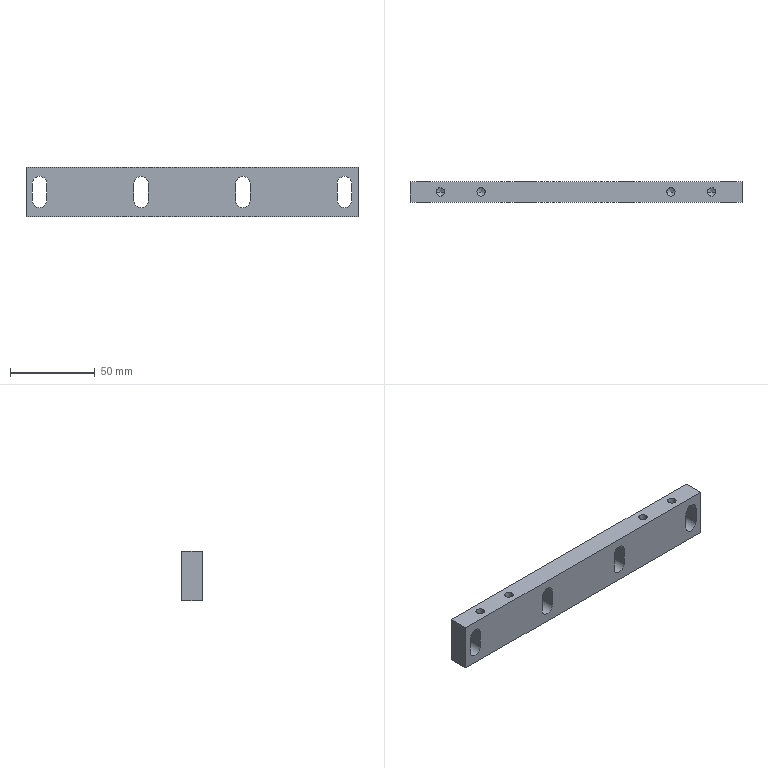Component | SolidWorks | 10AdjustmentPlate9.26-2 | 1 solid | 42 faces | box 196 x 12 x 29 mm | volume 59951 mm3 | cylinder 20 | plane 14 | cone 8 | commonest cylinder face diameters 8.5 x12 5 x8
build123d program:
from build123d import *

# Parameters (mm, degrees)
SKETCH1_W             = 196
SKETCH1_H             = 12
BOSS_EXTRUDE1_DEPTH   = 29
CUT_EXTRUDE1_DEPTH    = 199.497
M6_TAPPED_HOLE1_D     = 5
M6_TAPPED_HOLE1_DEPTH = 18
M6_TAPPED_HOLE1_TIP   = 1.502


with BuildPart() as part:
    # Sketch1 → Boss-Extrude1 (new body)
    with BuildSketch(Plane.XY):
        with Locations((98, -6)):
            Rectangle(SKETCH1_W, SKETCH1_H)
    extrude(amount=BOSS_EXTRUDE1_DEPTH)

    # Sketch2 → Cut-Extrude1 (cut, through all)
    with BuildSketch(Plane(origin=(0, 0, 0), x_dir=(1, 0, 0), z_dir=(0, 1, 0))):
        with BuildLine():
            Line((12.25, -9.5), (12.25, -19.5))
            ThreePointArc((12.25, -19.5), (8, -23.75), (3.75, -19.5))
            Line((3.75, -19.5), (3.75, -9.5))
            ThreePointArc((3.75, -9.5), (8, -5.25), (12.25, -9.5))
        make_face()
        with BuildLine():
            Line((72.25, -9.5), (72.25, -19.5))
            ThreePointArc((72.25, -19.5), (68, -23.75), (63.75, -19.5))
            Line((63.75, -19.5), (63.75, -9.5))
            ThreePointArc((63.75, -9.5), (68, -5.25), (72.25, -9.5))
        make_face()
        with BuildLine():
            Line((183.75, -9.5), (183.75, -19.5))
            ThreePointArc((183.75, -19.5), (188, -23.75), (192.25, -19.5))
            Line((192.25, -19.5), (192.25, -9.5))
            ThreePointArc((192.25, -9.5), (188, -5.25), (183.75, -9.5))
        make_face()
        with BuildLine():
            Line((123.75, -9.5), (123.75, -19.5))
            ThreePointArc((123.75, -19.5), (128, -23.75), (132.25, -19.5))
            Line((132.25, -19.5), (132.25, -9.5))
            ThreePointArc((132.25, -9.5), (128, -5.25), (123.75, -9.5))
        make_face()
    extrude(amount=-CUT_EXTRUDE1_DEPTH, mode=Mode.SUBTRACT)

    # M6 Tapped Hole1
    with Locations(Plane.XY.offset(29)):
        with Locations((18, -6), (42, -6), (178, -6), (154, -6)):
            Hole(M6_TAPPED_HOLE1_D / 2, depth=M6_TAPPED_HOLE1_DEPTH)
            with Locations((0, 0, -(M6_TAPPED_HOLE1_DEPTH + M6_TAPPED_HOLE1_TIP / 2))):  # 118° drill point
                Cone(0, M6_TAPPED_HOLE1_D / 2, M6_TAPPED_HOLE1_TIP, mode=Mode.SUBTRACT)


solid = part.part

# Placed as in the assembly
solid = solid.moved(Location((90, -163, -39), (0, 0, 0)))